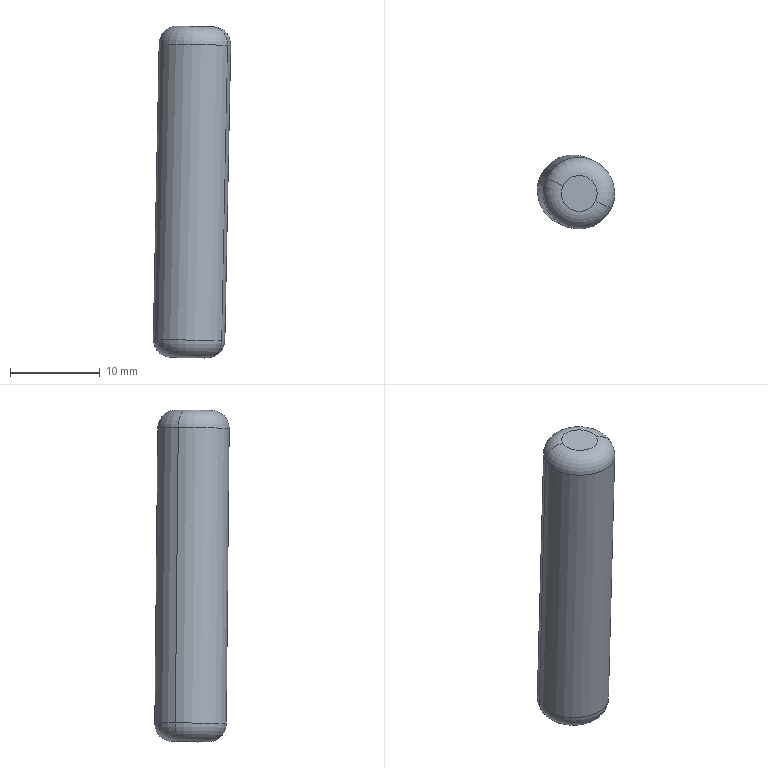Component | SolidWorks | VehicleRearAxis-1 | 1 solid | 8 faces | box 8.65 x 8.33 x 37.08 mm | volume 1821 mm3 | torus 4 | cylinder 2 | plane 2 | commonest cylinder face diameters 8 x2
build123d program:
from build123d import *

# Parameters (mm, degrees)
SKETCH1_R           = 4
BOSS_EXTRUDE1_DEPTH = 37
FILLET1_R           = 2


with BuildPart() as part:
    # Sketch1 → Boss-Extrude1 (new body)
    with BuildSketch(Plane.XY):
        with Locations((-20.298, -1.186)):
            Circle(SKETCH1_R)
    extrude(amount=BOSS_EXTRUDE1_DEPTH)

    # Fillet1
    fillet1_edges = [part.edges().sort_by_distance(p)[0] for p in [
        (-24.298, -1.186, 0),
        (-24.298, -1.186, 37),
    ]]
    fillet(fillet1_edges, radius=FILLET1_R)


solid = part.part

# Placed as in the assembly
solid = solid.moved(Location((-20.022, -23.96, -17.929), (0.5722, 1.137, -126.026)))
STEP:
#1=COLOUR_RGB('',0.7922,0.8196,0.9333);
#2=FILL_AREA_STYLE_COLOUR('',#1);
#3=FILL_AREA_STYLE('',(#2));
#4=SURFACE_STYLE_FILL_AREA(#3);
#5=SURFACE_SIDE_STYLE('',(#4));
#6=SURFACE_STYLE_USAGE(.BOTH.,#5);
#7=PRESENTATION_STYLE_ASSIGNMENT((#6));
#8=CARTESIAN_POINT('',(-0.4713,-0.2163,0.6734));
#9=VERTEX_POINT('',#8);
#10=CARTESIAN_POINT('',(-0.1862,-0.3501,0.6664));
#11=VERTEX_POINT('',#10);
#12=CARTESIAN_POINT('',(-0.3288,-0.2832,0.6699));
#13=DIRECTION('',(-0.01984,0.009985,-0.9998));
#14=DIRECTION('',(0.905,-0.4248,-0.0222));
#15=AXIS2_PLACEMENT_3D('',#12,#13,#14);
#16=CIRCLE('',#15,0.1575);
#17=EDGE_CURVE('',#9,#11,#16,.T.);
#18=ORIENTED_EDGE('',*,*,#17,.F.);
#19=CARTESIAN_POINT('',(-0.3985,-0.2506,0.7504));
#20=VERTEX_POINT('',#19);
#21=CARTESIAN_POINT('',(-0.4,-0.2498,0.6716));
#22=DIRECTION('',(0.4249,0.9052,0.0006096));
#23=DIRECTION('',(-0.9052,0.4249,0.));
#24=AXIS2_PLACEMENT_3D('',#21,#22,#23);
#25=CIRCLE('',#24,0.07874);
#26=EDGE_CURVE('',#9,#20,#25,.T.);
#27=ORIENTED_EDGE('',*,*,#26,.T.);
#28=CARTESIAN_POINT('',(-0.2559,-0.3175,0.7469));
#29=VERTEX_POINT('',#28);
#30=CARTESIAN_POINT('',(-0.3272,-0.284,0.7486));
#31=DIRECTION('',(0.01984,-0.009985,0.9998));
#32=DIRECTION('',(0.905,-0.4248,-0.0222));
#33=AXIS2_PLACEMENT_3D('',#30,#31,#32);
#34=CIRCLE('',#33,0.07874);
#35=EDGE_CURVE('',#29,#20,#34,.T.);
#36=ORIENTED_EDGE('',*,*,#35,.F.);
#37=CARTESIAN_POINT('',(-0.2575,-0.3167,0.6681));
#38=DIRECTION('',(-0.4249,-0.9052,-0.0006096));
#39=DIRECTION('',(0.9052,-0.4249,0.));
#40=AXIS2_PLACEMENT_3D('',#37,#38,#39);
#41=CIRCLE('',#40,0.07874);
#42=EDGE_CURVE('',#11,#29,#41,.T.);
#43=ORIENTED_EDGE('',*,*,#42,.F.);
#44=EDGE_LOOP('',(#18,#27,#36,#43));
#45=FACE_OUTER_BOUND('',#44,.T.);
#46=CARTESIAN_POINT('',(-0.3288,-0.2832,0.6699));
#47=DIRECTION('',(0.01984,-0.009985,0.9998));
#48=DIRECTION('',(0.905,-0.4248,-0.0222));
#49=AXIS2_PLACEMENT_3D('',#46,#47,#48);
#50=TOROIDAL_SURFACE('',#49,0.07874,0.07874);
#51=ADVANCED_FACE('',(#45),#50,.T.);
#52=CARTESIAN_POINT('',(-0.4274,-0.236,-0.706));
#53=VERTEX_POINT('',#52);
#54=CARTESIAN_POINT('',(-0.2848,-0.3029,-0.7095));
#55=VERTEX_POINT('',#54);
#56=CARTESIAN_POINT('',(-0.3561,-0.2695,-0.7077));
#57=DIRECTION('',(-0.01984,0.009985,-0.9998));
#58=DIRECTION('',(0.905,-0.4248,-0.0222));
#59=AXIS2_PLACEMENT_3D('',#56,#57,#58);
#60=CIRCLE('',#59,0.07874);
#61=EDGE_CURVE('',#53,#55,#60,.T.);
#62=ORIENTED_EDGE('',*,*,#61,.F.);
#63=CARTESIAN_POINT('',(-0.4971,-0.2034,-0.6255));
#64=VERTEX_POINT('',#63);
#65=CARTESIAN_POINT('',(-0.4258,-0.2368,-0.6272));
#66=DIRECTION('',(0.4249,0.9052,0.0006096));
#67=DIRECTION('',(-0.9052,0.4249,0.));
#68=AXIS2_PLACEMENT_3D('',#65,#66,#67);
#69=CIRCLE('',#68,0.07874);
#70=EDGE_CURVE('',#53,#64,#69,.T.);
#71=ORIENTED_EDGE('',*,*,#70,.T.);
#72=CARTESIAN_POINT('',(-0.212,-0.3372,-0.6325));
#73=VERTEX_POINT('',#72);
#74=CARTESIAN_POINT('',(-0.3545,-0.2703,-0.629));
#75=DIRECTION('',(0.01984,-0.009985,0.9998));
#76=DIRECTION('',(0.905,-0.4248,-0.0222));
#77=AXIS2_PLACEMENT_3D('',#74,#75,#76);
#78=CIRCLE('',#77,0.1575);
#79=EDGE_CURVE('',#73,#64,#78,.T.);
#80=ORIENTED_EDGE('',*,*,#79,.F.);
#81=CARTESIAN_POINT('',(-0.2833,-0.3037,-0.6307));
#82=DIRECTION('',(-0.4249,-0.9052,-0.0006096));
#83=DIRECTION('',(0.9052,-0.4249,0.));
#84=AXIS2_PLACEMENT_3D('',#81,#82,#83);
#85=CIRCLE('',#84,0.07874);
#86=EDGE_CURVE('',#55,#73,#85,.T.);
#87=ORIENTED_EDGE('',*,*,#86,.F.);
#88=EDGE_LOOP('',(#62,#71,#80,#87));
#89=FACE_OUTER_BOUND('',#88,.T.);
#90=CARTESIAN_POINT('',(-0.3545,-0.2703,-0.629));
#91=DIRECTION('',(0.01984,-0.009985,0.9998));
#92=DIRECTION('',(0.905,-0.4248,-0.0222));
#93=AXIS2_PLACEMENT_3D('',#90,#91,#92);
#94=TOROIDAL_SURFACE('',#93,0.07874,0.07874);
#95=ADVANCED_FACE('',(#89),#94,.T.);
#96=ORIENTED_EDGE('',*,*,#17,.T.);
#97=CARTESIAN_POINT('',(-0.1847,-0.3509,0.7451));
#98=DIRECTION('',(-0.01984,0.009985,-0.9998));
#99=VECTOR('',#98,39.37);
#100=LINE('',#97,#99);
#101=EDGE_CURVE('',#11,#73,#100,.T.);
#102=ORIENTED_EDGE('',*,*,#101,.T.);
#103=ORIENTED_EDGE('',*,*,#79,.T.);
#104=CARTESIAN_POINT('',(-0.4697,-0.2171,0.7521));
#105=DIRECTION('',(-0.01984,0.009985,-0.9998));
#106=VECTOR('',#105,39.37);
#107=LINE('',#104,#106);
#108=EDGE_CURVE('',#9,#64,#107,.T.);
#109=ORIENTED_EDGE('',*,*,#108,.F.);
#110=EDGE_LOOP('',(#96,#102,#103,#109));
#111=FACE_OUTER_BOUND('',#110,.T.);
#112=CARTESIAN_POINT('',(-0.3272,-0.284,0.7486));
#113=DIRECTION('',(-0.01984,0.009985,-0.9998));
#114=DIRECTION('',(-0.905,0.4248,0.0222));
#115=AXIS2_PLACEMENT_3D('',#112,#113,#114);
#116=CYLINDRICAL_SURFACE('',#115,0.1575);
#117=ADVANCED_FACE('',(#111),#116,.T.);
#118=ORIENTED_EDGE('',*,*,#101,.F.);
#119=CARTESIAN_POINT('',(-0.3288,-0.2832,0.6699));
#120=DIRECTION('',(-0.01984,0.009985,-0.9998));
#121=DIRECTION('',(0.905,-0.4248,-0.0222));
#122=AXIS2_PLACEMENT_3D('',#119,#120,#121);
#123=CIRCLE('',#122,0.1575);
#124=EDGE_CURVE('',#11,#9,#123,.T.);
#125=ORIENTED_EDGE('',*,*,#124,.T.);
#126=ORIENTED_EDGE('',*,*,#108,.T.);
#127=CARTESIAN_POINT('',(-0.3545,-0.2703,-0.629));
#128=DIRECTION('',(0.01984,-0.009985,0.9998));
#129=DIRECTION('',(0.905,-0.4248,-0.0222));
#130=AXIS2_PLACEMENT_3D('',#127,#128,#129);
#131=CIRCLE('',#130,0.1575);
#132=EDGE_CURVE('',#64,#73,#131,.T.);
#133=ORIENTED_EDGE('',*,*,#132,.T.);
#134=EDGE_LOOP('',(#118,#125,#126,#133));
#135=FACE_OUTER_BOUND('',#134,.T.);
#136=CARTESIAN_POINT('',(-0.3272,-0.284,0.7486));
#137=DIRECTION('',(-0.01984,0.009985,-0.9998));
#138=DIRECTION('',(-0.905,0.4248,0.0222));
#139=AXIS2_PLACEMENT_3D('',#136,#137,#138);
#140=CYLINDRICAL_SURFACE('',#139,0.1575);
#141=ADVANCED_FACE('',(#135),#140,.T.);
#142=ORIENTED_EDGE('',*,*,#35,.T.);
#143=CARTESIAN_POINT('',(-0.3272,-0.284,0.7486));
#144=DIRECTION('',(0.01984,-0.009985,0.9998));
#145=DIRECTION('',(0.905,-0.4248,-0.0222));
#146=AXIS2_PLACEMENT_3D('',#143,#144,#145);
#147=CIRCLE('',#146,0.07874);
#148=EDGE_CURVE('',#20,#29,#147,.T.);
#149=ORIENTED_EDGE('',*,*,#148,.T.);
#150=EDGE_LOOP('',(#142,#149));
#151=FACE_OUTER_BOUND('',#150,.T.);
#152=CARTESIAN_POINT('',(-0.3272,-0.284,0.7486));
#153=DIRECTION('',(0.01984,-0.009985,0.9998));
#154=DIRECTION('',(0.905,-0.4248,-0.0222));
#155=AXIS2_PLACEMENT_3D('',#152,#153,#154);
#156=PLANE('',#155);
#157=ADVANCED_FACE('',(#151),#156,.T.);
#158=CARTESIAN_POINT('',(-0.3561,-0.2695,-0.7077));
#159=DIRECTION('',(-0.01984,0.009985,-0.9998));
#160=DIRECTION('',(0.905,-0.4248,-0.0222));
#161=AXIS2_PLACEMENT_3D('',#158,#159,#160);
#162=CIRCLE('',#161,0.07874);
#163=EDGE_CURVE('',#55,#53,#162,.T.);
#164=ORIENTED_EDGE('',*,*,#163,.T.);
#165=ORIENTED_EDGE('',*,*,#61,.T.);
#166=EDGE_LOOP('',(#164,#165));
#167=FACE_OUTER_BOUND('',#166,.T.);
#168=CARTESIAN_POINT('',(-0.3561,-0.2695,-0.7077));
#169=DIRECTION('',(0.01984,-0.009985,0.9998));
#170=DIRECTION('',(0.905,-0.4248,-0.0222));
#171=AXIS2_PLACEMENT_3D('',#168,#169,#170);
#172=PLANE('',#171);
#173=ADVANCED_FACE('',(#167),#172,.F.);
#174=ORIENTED_EDGE('',*,*,#70,.F.);
#175=ORIENTED_EDGE('',*,*,#163,.F.);
#176=ORIENTED_EDGE('',*,*,#86,.T.);
#177=ORIENTED_EDGE('',*,*,#132,.F.);
#178=EDGE_LOOP('',(#174,#175,#176,#177));
#179=FACE_OUTER_BOUND('',#178,.T.);
#180=CARTESIAN_POINT('',(-0.3545,-0.2703,-0.629));
#181=DIRECTION('',(0.01984,-0.009985,0.9998));
#182=DIRECTION('',(0.905,-0.4248,-0.0222));
#183=AXIS2_PLACEMENT_3D('',#180,#181,#182);
#184=TOROIDAL_SURFACE('',#183,0.07874,0.07874);
#185=ADVANCED_FACE('',(#179),#184,.T.);
#186=ORIENTED_EDGE('',*,*,#26,.F.);
#187=ORIENTED_EDGE('',*,*,#124,.F.);
#188=ORIENTED_EDGE('',*,*,#42,.T.);
#189=ORIENTED_EDGE('',*,*,#148,.F.);
#190=EDGE_LOOP('',(#186,#187,#188,#189));
#191=FACE_OUTER_BOUND('',#190,.T.);
#192=CARTESIAN_POINT('',(-0.3288,-0.2832,0.6699));
#193=DIRECTION('',(0.01984,-0.009985,0.9998));
#194=DIRECTION('',(0.905,-0.4248,-0.0222));
#195=AXIS2_PLACEMENT_3D('',#192,#193,#194);
#196=TOROIDAL_SURFACE('',#195,0.07874,0.07874);
#197=ADVANCED_FACE('',(#191),#196,.T.);
#198=CLOSED_SHELL('',(#51,#95,#117,#141,#157,#173,#185,#197));
#199=MANIFOLD_SOLID_BREP('',#198);
#200=STYLED_ITEM('',(#7),#199);
#201=PRESENTATION_LAYER_ASSIGNMENT('','',(#200));
#202=CARTESIAN_POINT('',(0.,0.,0.));
#203=DIRECTION('',(0.,0.,1.));
#204=DIRECTION('',(1.,0.,0.));
#205=AXIS2_PLACEMENT_3D('',#202,#203,#204);
#206=(LENGTH_UNIT()NAMED_UNIT(*)SI_UNIT($,.METRE.));
#207=LENGTH_MEASURE_WITH_UNIT(LENGTH_MEASURE(0.0254),#206);
#208=DIMENSIONAL_EXPONENTS(1.,0.,0.,0.,0.,0.,0.);
#209=(CONVERSION_BASED_UNIT('',#207)LENGTH_UNIT()NAMED_UNIT(#208));
#210=UNCERTAINTY_MEASURE_WITH_UNIT(LENGTH_MEASURE(0.00001),#209,'','');
#211=(NAMED_UNIT(*)PLANE_ANGLE_UNIT()SI_UNIT($,.RADIAN.));
#212=(NAMED_UNIT(*)SI_UNIT($,.STERADIAN.)SOLID_ANGLE_UNIT());
#213=(GEOMETRIC_REPRESENTATION_CONTEXT(3)GLOBAL_UNCERTAINTY_ASSIGNED_CONTEXT((#210))GLOBAL_UNIT_ASSIGNED_CONTEXT((#209,#211,#212))REPRESENTATION_CONTEXT('',''));
#214=ADVANCED_BREP_SHAPE_REPRESENTATION('',(#199,#205),#213);
#215=(LENGTH_UNIT()NAMED_UNIT(*)SI_UNIT($,.METRE.));
#216=LENGTH_MEASURE_WITH_UNIT(LENGTH_MEASURE(0.0254),#215);
#217=DIMENSIONAL_EXPONENTS(1.,0.,0.,0.,0.,0.,0.);
#218=(CONVERSION_BASED_UNIT('',#216)LENGTH_UNIT()NAMED_UNIT(#217));
#219=UNCERTAINTY_MEASURE_WITH_UNIT(LENGTH_MEASURE(0.00001),#218,'','');
#220=(NAMED_UNIT(*)PLANE_ANGLE_UNIT()SI_UNIT($,.RADIAN.));
#221=(NAMED_UNIT(*)SI_UNIT($,.STERADIAN.)SOLID_ANGLE_UNIT());
#222=(GEOMETRIC_REPRESENTATION_CONTEXT(3)GLOBAL_UNCERTAINTY_ASSIGNED_CONTEXT((#219))GLOBAL_UNIT_ASSIGNED_CONTEXT((#218,#220,#221))REPRESENTATION_CONTEXT('',''));
#223=MECHANICAL_DESIGN_GEOMETRIC_PRESENTATION_REPRESENTATION('',(#200),#222);